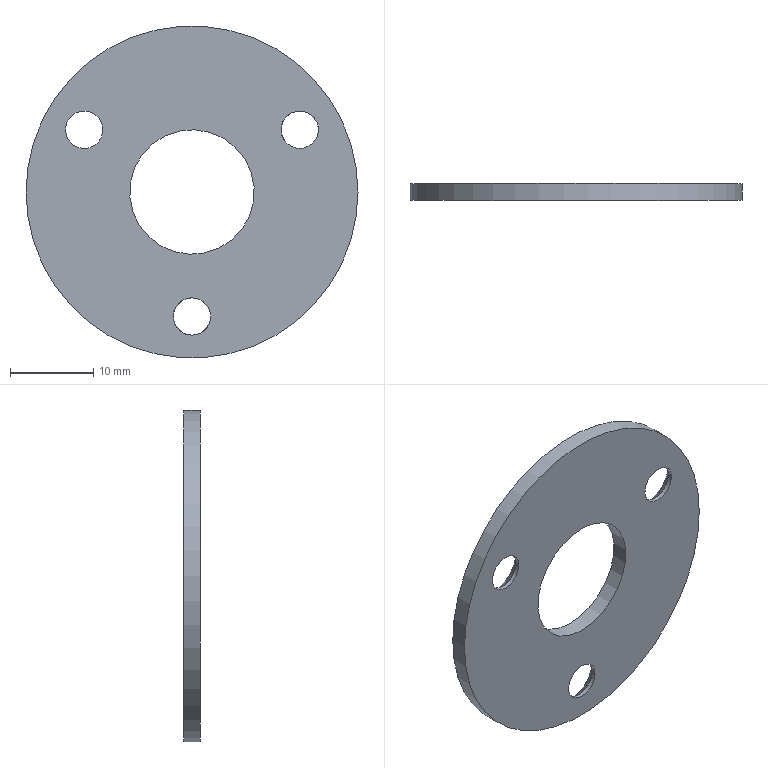Component | NX | GLAND | 1 solid | 10 faces | box 40 x 2 x 40 mm | volume 2006 mm3 | cylinder 5 | cone 3 | plane 2 | commonest cylinder face diameters 4.5 x3 15 x1 40 x1
STEP:
#1=CARTESIAN_POINT('',(0.,0.,0.));
#2=DIRECTION('',(0.,0.,1.));
#3=DIRECTION('',(1.,0.,0.));
#4=AXIS2_PLACEMENT_3D('',#1,#2,#3);
#5=CARTESIAN_POINT('',(3.75,36.,10.995));
#6=VERTEX_POINT('',#5);
#7=CARTESIAN_POINT('',(-0.,36.,4.5));
#8=DIRECTION('',(0.,-1.,0.));
#9=DIRECTION('',(0.5,0.,0.866));
#10=AXIS2_PLACEMENT_3D('',#7,#8,#9);
#11=CIRCLE('',#10,7.5);
#12=CARTESIAN_POINT('',(-0.,36.,4.5));
#13=DIRECTION('',(0.,-1.,0.));
#14=DIRECTION('',(-0.5,0.,-0.866));
#15=AXIS2_PLACEMENT_3D('',#12,#13,#14);
#16=CYLINDRICAL_SURFACE('',#15,7.5);
#17=CARTESIAN_POINT('',(3.142,0.));
#18=DIRECTION('',(1.,0.));
#19=VECTOR('',#18,1.);
#20=LINE('',#17,#19);
#21=(GEOMETRIC_REPRESENTATION_CONTEXT(2)PARAMETRIC_REPRESENTATION_CONTEXT()REPRESENTATION_CONTEXT('',''));
#22=DEFINITIONAL_REPRESENTATION('',(#20),#21);
#23=PCURVE('',#16,#22);
#24=CARTESIAN_POINT('',(-6.495,36.,8.25));
#25=DIRECTION('',(0.,-1.,0.));
#26=DIRECTION('',(-0.5,0.,-0.866));
#27=AXIS2_PLACEMENT_3D('',#24,#25,#26);
#28=PLANE('',#27);
#29=CARTESIAN_POINT('',(-0.,7.5));
#30=DIRECTION('',(-1.,0.));
#31=AXIS2_PLACEMENT_2D('',#29,#30);
#32=CIRCLE('',#31,7.5);
#33=(GEOMETRIC_REPRESENTATION_CONTEXT(2)PARAMETRIC_REPRESENTATION_CONTEXT()REPRESENTATION_CONTEXT('',''));
#34=DEFINITIONAL_REPRESENTATION('',(#32),#33);
#35=PCURVE('',#28,#34);
#36=SURFACE_CURVE('',#11,(#23,#35),.PCURVE_S1.);
#37=EDGE_CURVE('',#6,#6,#36,.T.);
#38=ORIENTED_EDGE('',*,*,#37,.T.);
#39=CARTESIAN_POINT('',(3.75,34.,10.995));
#40=VERTEX_POINT('',#39);
#41=CARTESIAN_POINT('',(3.75,36.,10.995));
#42=CARTESIAN_POINT('',(3.75,34.,10.995));
#43=B_SPLINE_CURVE_WITH_KNOTS('',1,(#41,#42),.UNSPECIFIED.,.F.,.F.,(2,2),(0.,2.),.PIECEWISE_BEZIER_KNOTS.);
#44=CARTESIAN_POINT('',(9.425,0.));
#45=DIRECTION('',(0.,1.));
#46=VECTOR('',#45,1.);
#47=LINE('',#44,#46);
#48=(GEOMETRIC_REPRESENTATION_CONTEXT(2)PARAMETRIC_REPRESENTATION_CONTEXT()REPRESENTATION_CONTEXT('',''));
#49=DEFINITIONAL_REPRESENTATION('',(#47),#48);
#50=PCURVE('',#16,#49);
#51=CARTESIAN_POINT('',(3.142,0.));
#52=DIRECTION('',(0.,1.));
#53=VECTOR('',#52,1.);
#54=LINE('',#51,#53);
#55=(GEOMETRIC_REPRESENTATION_CONTEXT(2)PARAMETRIC_REPRESENTATION_CONTEXT()REPRESENTATION_CONTEXT('',''));
#56=DEFINITIONAL_REPRESENTATION('',(#54),#55);
#57=PCURVE('',#16,#56);
#58=SEAM_CURVE('',#43,(#50,#57),.PCURVE_S1.);
#59=EDGE_CURVE('',#6,#40,#58,.T.);
#60=ORIENTED_EDGE('',*,*,#59,.T.);
#61=CARTESIAN_POINT('',(-0.,34.,4.5));
#62=DIRECTION('',(0.,-1.,0.));
#63=DIRECTION('',(0.5,0.,0.866));
#64=AXIS2_PLACEMENT_3D('',#61,#62,#63);
#65=CIRCLE('',#64,7.5);
#66=CARTESIAN_POINT('',(3.142,2.));
#67=DIRECTION('',(1.,0.));
#68=VECTOR('',#67,1.);
#69=LINE('',#66,#68);
#70=(GEOMETRIC_REPRESENTATION_CONTEXT(2)PARAMETRIC_REPRESENTATION_CONTEXT()REPRESENTATION_CONTEXT('',''));
#71=DEFINITIONAL_REPRESENTATION('',(#69),#70);
#72=PCURVE('',#16,#71);
#73=CARTESIAN_POINT('',(-6.495,34.,8.25));
#74=DIRECTION('',(0.,-1.,0.));
#75=DIRECTION('',(-0.5,0.,-0.866));
#76=AXIS2_PLACEMENT_3D('',#73,#74,#75);
#77=PLANE('',#76);
#78=CARTESIAN_POINT('',(-0.,7.5));
#79=DIRECTION('',(-1.,0.));
#80=AXIS2_PLACEMENT_2D('',#78,#79);
#81=CIRCLE('',#80,7.5);
#82=(GEOMETRIC_REPRESENTATION_CONTEXT(2)PARAMETRIC_REPRESENTATION_CONTEXT()REPRESENTATION_CONTEXT('',''));
#83=DEFINITIONAL_REPRESENTATION('',(#81),#82);
#84=PCURVE('',#77,#83);
#85=SURFACE_CURVE('',#65,(#72,#84),.PCURVE_S1.);
#86=EDGE_CURVE('',#40,#40,#85,.T.);
#87=ORIENTED_EDGE('',*,*,#86,.F.);
#88=ORIENTED_EDGE('',*,*,#59,.F.);
#89=EDGE_LOOP('',(#38,#60,#87,#88));
#90=FACE_BOUND('',#89,.F.);
#91=ADVANCED_FACE('',(#90),#16,.F.);
#92=CARTESIAN_POINT('',(-1.125,34.5,-12.449));
#93=VERTEX_POINT('',#92);
#94=CARTESIAN_POINT('',(0.,34.5,-10.5));
#95=DIRECTION('',(0.,1.,0.));
#96=DIRECTION('',(-0.5,0.,-0.866));
#97=AXIS2_PLACEMENT_3D('',#94,#95,#96);
#98=CIRCLE('',#97,2.25);
#99=CARTESIAN_POINT('',(0.,36.,-10.5));
#100=DIRECTION('',(0.,-1.,0.));
#101=DIRECTION('',(-0.5,0.,-0.866));
#102=AXIS2_PLACEMENT_3D('',#99,#100,#101);
#103=CYLINDRICAL_SURFACE('',#102,2.25);
#104=CARTESIAN_POINT('',(6.283,1.5));
#105=DIRECTION('',(-1.,0.));
#106=VECTOR('',#105,1.);
#107=LINE('',#104,#106);
#108=(GEOMETRIC_REPRESENTATION_CONTEXT(2)PARAMETRIC_REPRESENTATION_CONTEXT()REPRESENTATION_CONTEXT('',''));
#109=DEFINITIONAL_REPRESENTATION('',(#107),#108);
#110=PCURVE('',#103,#109);
#111=CARTESIAN_POINT('',(0.,36.,-10.5));
#112=DIRECTION('',(0.,1.,0.));
#113=DIRECTION('',(0.5,0.,0.866));
#114=AXIS2_PLACEMENT_3D('',#111,#112,#113);
#115=CONICAL_SURFACE('',#114,3.75,0.7854);
#116=CARTESIAN_POINT('',(3.142,-1.5));
#117=DIRECTION('',(1.,0.));
#118=VECTOR('',#117,1.);
#119=LINE('',#116,#118);
#120=(GEOMETRIC_REPRESENTATION_CONTEXT(2)PARAMETRIC_REPRESENTATION_CONTEXT()REPRESENTATION_CONTEXT('',''));
#121=DEFINITIONAL_REPRESENTATION('',(#119),#120);
#122=PCURVE('',#115,#121);
#123=SURFACE_CURVE('',#98,(#110,#122),.PCURVE_S1.);
#124=EDGE_CURVE('',#93,#93,#123,.T.);
#125=ORIENTED_EDGE('',*,*,#124,.F.);
#126=CARTESIAN_POINT('',(-1.125,34.,-12.449));
#127=VERTEX_POINT('',#126);
#128=CARTESIAN_POINT('',(-1.125,34.5,-12.449));
#129=CARTESIAN_POINT('',(-1.125,34.,-12.449));
#130=B_SPLINE_CURVE_WITH_KNOTS('',1,(#128,#129),.UNSPECIFIED.,.F.,.F.,(2,2),(1.5,2.),.PIECEWISE_BEZIER_KNOTS.);
#131=CARTESIAN_POINT('',(6.283,0.));
#132=DIRECTION('',(0.,1.));
#133=VECTOR('',#132,1.);
#134=LINE('',#131,#133);
#135=(GEOMETRIC_REPRESENTATION_CONTEXT(2)PARAMETRIC_REPRESENTATION_CONTEXT()REPRESENTATION_CONTEXT('',''));
#136=DEFINITIONAL_REPRESENTATION('',(#134),#135);
#137=PCURVE('',#103,#136);
#138=CARTESIAN_POINT('',(0.,0.));
#139=DIRECTION('',(0.,1.));
#140=VECTOR('',#139,1.);
#141=LINE('',#138,#140);
#142=(GEOMETRIC_REPRESENTATION_CONTEXT(2)PARAMETRIC_REPRESENTATION_CONTEXT()REPRESENTATION_CONTEXT('',''));
#143=DEFINITIONAL_REPRESENTATION('',(#141),#142);
#144=PCURVE('',#103,#143);
#145=SEAM_CURVE('',#130,(#137,#144),.PCURVE_S1.);
#146=EDGE_CURVE('',#93,#127,#145,.T.);
#147=ORIENTED_EDGE('',*,*,#146,.T.);
#148=CARTESIAN_POINT('',(-2.25,34.,-10.5));
#149=VERTEX_POINT('',#148);
#150=CARTESIAN_POINT('',(0.,34.,-10.5));
#151=DIRECTION('',(0.,-1.,0.));
#152=DIRECTION('',(-1.,0.,-0.));
#153=AXIS2_PLACEMENT_3D('',#150,#151,#152);
#154=CIRCLE('',#153,2.25);
#155=CARTESIAN_POINT('',(5.236,2.));
#156=DIRECTION('',(1.,0.));
#157=VECTOR('',#156,1.);
#158=LINE('',#155,#157);
#159=(GEOMETRIC_REPRESENTATION_CONTEXT(2)PARAMETRIC_REPRESENTATION_CONTEXT()REPRESENTATION_CONTEXT('',''));
#160=DEFINITIONAL_REPRESENTATION('',(#158),#159);
#161=PCURVE('',#103,#160);
#162=CARTESIAN_POINT('',(12.99,15.));
#163=DIRECTION('',(0.5,-0.866));
#164=AXIS2_PLACEMENT_2D('',#162,#163);
#165=CIRCLE('',#164,2.25);
#166=(GEOMETRIC_REPRESENTATION_CONTEXT(2)PARAMETRIC_REPRESENTATION_CONTEXT()REPRESENTATION_CONTEXT('',''));
#167=DEFINITIONAL_REPRESENTATION('',(#165),#166);
#168=PCURVE('',#77,#167);
#169=SURFACE_CURVE('',#154,(#161,#168),.PCURVE_S1.);
#170=EDGE_CURVE('',#149,#127,#169,.T.);
#171=ORIENTED_EDGE('',*,*,#170,.F.);
#172=CARTESIAN_POINT('',(0.,34.,-10.5));
#173=DIRECTION('',(0.,-1.,0.));
#174=DIRECTION('',(-1.,0.,-0.));
#175=AXIS2_PLACEMENT_3D('',#172,#173,#174);
#176=CIRCLE('',#175,2.25);
#177=CARTESIAN_POINT('',(-1.047,2.));
#178=DIRECTION('',(1.,0.));
#179=VECTOR('',#178,1.);
#180=LINE('',#177,#179);
#181=(GEOMETRIC_REPRESENTATION_CONTEXT(2)PARAMETRIC_REPRESENTATION_CONTEXT()REPRESENTATION_CONTEXT('',''));
#182=DEFINITIONAL_REPRESENTATION('',(#180),#181);
#183=PCURVE('',#103,#182);
#184=CARTESIAN_POINT('',(12.99,15.));
#185=DIRECTION('',(0.5,-0.866));
#186=AXIS2_PLACEMENT_2D('',#184,#185);
#187=CIRCLE('',#186,2.25);
#188=(GEOMETRIC_REPRESENTATION_CONTEXT(2)PARAMETRIC_REPRESENTATION_CONTEXT()REPRESENTATION_CONTEXT('',''));
#189=DEFINITIONAL_REPRESENTATION('',(#187),#188);
#190=PCURVE('',#77,#189);
#191=SURFACE_CURVE('',#176,(#183,#190),.PCURVE_S1.);
#192=EDGE_CURVE('',#127,#149,#191,.T.);
#193=ORIENTED_EDGE('',*,*,#192,.F.);
#194=ORIENTED_EDGE('',*,*,#146,.F.);
#195=EDGE_LOOP('',(#125,#147,#171,#193,#194));
#196=FACE_BOUND('',#195,.F.);
#197=ADVANCED_FACE('',(#196),#103,.F.);
#198=CARTESIAN_POINT('',(-14.115,34.5,10.051));
#199=VERTEX_POINT('',#198);
#200=CARTESIAN_POINT('',(-12.99,34.5,12.));
#201=DIRECTION('',(0.,1.,0.));
#202=DIRECTION('',(-0.5,0.,-0.866));
#203=AXIS2_PLACEMENT_3D('',#200,#201,#202);
#204=CIRCLE('',#203,2.25);
#205=CARTESIAN_POINT('',(-12.99,36.,12.));
#206=DIRECTION('',(0.,-1.,0.));
#207=DIRECTION('',(-0.5,0.,-0.866));
#208=AXIS2_PLACEMENT_3D('',#205,#206,#207);
#209=CYLINDRICAL_SURFACE('',#208,2.25);
#210=CARTESIAN_POINT('',(6.283,1.5));
#211=DIRECTION('',(-1.,0.));
#212=VECTOR('',#211,1.);
#213=LINE('',#210,#212);
#214=(GEOMETRIC_REPRESENTATION_CONTEXT(2)PARAMETRIC_REPRESENTATION_CONTEXT()REPRESENTATION_CONTEXT('',''));
#215=DEFINITIONAL_REPRESENTATION('',(#213),#214);
#216=PCURVE('',#209,#215);
#217=CARTESIAN_POINT('',(-12.99,36.,12.));
#218=DIRECTION('',(0.,1.,0.));
#219=DIRECTION('',(0.5,0.,0.866));
#220=AXIS2_PLACEMENT_3D('',#217,#218,#219);
#221=CONICAL_SURFACE('',#220,3.75,0.7854);
#222=CARTESIAN_POINT('',(3.142,-1.5));
#223=DIRECTION('',(1.,0.));
#224=VECTOR('',#223,1.);
#225=LINE('',#222,#224);
#226=(GEOMETRIC_REPRESENTATION_CONTEXT(2)PARAMETRIC_REPRESENTATION_CONTEXT()REPRESENTATION_CONTEXT('',''));
#227=DEFINITIONAL_REPRESENTATION('',(#225),#226);
#228=PCURVE('',#221,#227);
#229=SURFACE_CURVE('',#204,(#216,#228),.PCURVE_S1.);
#230=EDGE_CURVE('',#199,#199,#229,.T.);
#231=ORIENTED_EDGE('',*,*,#230,.F.);
#232=CARTESIAN_POINT('',(-14.115,34.,10.051));
#233=VERTEX_POINT('',#232);
#234=CARTESIAN_POINT('',(-14.115,34.5,10.051));
#235=CARTESIAN_POINT('',(-14.115,34.,10.051));
#236=B_SPLINE_CURVE_WITH_KNOTS('',1,(#234,#235),.UNSPECIFIED.,.F.,.F.,(2,2),(1.5,2.),.PIECEWISE_BEZIER_KNOTS.);
#237=CARTESIAN_POINT('',(6.283,0.));
#238=DIRECTION('',(0.,1.));
#239=VECTOR('',#238,1.);
#240=LINE('',#237,#239);
#241=(GEOMETRIC_REPRESENTATION_CONTEXT(2)PARAMETRIC_REPRESENTATION_CONTEXT()REPRESENTATION_CONTEXT('',''));
#242=DEFINITIONAL_REPRESENTATION('',(#240),#241);
#243=PCURVE('',#209,#242);
#244=CARTESIAN_POINT('',(0.,0.));
#245=DIRECTION('',(0.,1.));
#246=VECTOR('',#245,1.);
#247=LINE('',#244,#246);
#248=(GEOMETRIC_REPRESENTATION_CONTEXT(2)PARAMETRIC_REPRESENTATION_CONTEXT()REPRESENTATION_CONTEXT('',''));
#249=DEFINITIONAL_REPRESENTATION('',(#247),#248);
#250=PCURVE('',#209,#249);
#251=SEAM_CURVE('',#236,(#243,#250),.PCURVE_S1.);
#252=EDGE_CURVE('',#199,#233,#251,.T.);
#253=ORIENTED_EDGE('',*,*,#252,.T.);
#254=CARTESIAN_POINT('',(-11.865,34.,13.949));
#255=VERTEX_POINT('',#254);
#256=CARTESIAN_POINT('',(-12.99,34.,12.));
#257=DIRECTION('',(0.,-1.,0.));
#258=DIRECTION('',(0.5,0.,0.866));
#259=AXIS2_PLACEMENT_3D('',#256,#257,#258);
#260=CIRCLE('',#259,2.25);
#261=CARTESIAN_POINT('',(3.142,2.));
#262=DIRECTION('',(1.,0.));
#263=VECTOR('',#262,1.);
#264=LINE('',#261,#263);
#265=(GEOMETRIC_REPRESENTATION_CONTEXT(2)PARAMETRIC_REPRESENTATION_CONTEXT()REPRESENTATION_CONTEXT('',''));
#266=DEFINITIONAL_REPRESENTATION('',(#264),#265);
#267=PCURVE('',#209,#266);
#268=CARTESIAN_POINT('',(-0.,-7.5));
#269=DIRECTION('',(-1.,0.));
#270=AXIS2_PLACEMENT_2D('',#268,#269);
#271=CIRCLE('',#270,2.25);
#272=(GEOMETRIC_REPRESENTATION_CONTEXT(2)PARAMETRIC_REPRESENTATION_CONTEXT()REPRESENTATION_CONTEXT('',''));
#273=DEFINITIONAL_REPRESENTATION('',(#271),#272);
#274=PCURVE('',#77,#273);
#275=SURFACE_CURVE('',#260,(#267,#274),.PCURVE_S1.);
#276=EDGE_CURVE('',#255,#233,#275,.T.);
#277=ORIENTED_EDGE('',*,*,#276,.F.);
#278=CARTESIAN_POINT('',(-12.99,34.,12.));
#279=DIRECTION('',(0.,-1.,0.));
#280=DIRECTION('',(0.5,0.,0.866));
#281=AXIS2_PLACEMENT_3D('',#278,#279,#280);
#282=CIRCLE('',#281,2.25);
#283=CARTESIAN_POINT('',(-3.142,2.));
#284=DIRECTION('',(1.,0.));
#285=VECTOR('',#284,1.);
#286=LINE('',#283,#285);
#287=(GEOMETRIC_REPRESENTATION_CONTEXT(2)PARAMETRIC_REPRESENTATION_CONTEXT()REPRESENTATION_CONTEXT('',''));
#288=DEFINITIONAL_REPRESENTATION('',(#286),#287);
#289=PCURVE('',#209,#288);
#290=CARTESIAN_POINT('',(-0.,-7.5));
#291=DIRECTION('',(-1.,0.));
#292=AXIS2_PLACEMENT_2D('',#290,#291);
#293=CIRCLE('',#292,2.25);
#294=(GEOMETRIC_REPRESENTATION_CONTEXT(2)PARAMETRIC_REPRESENTATION_CONTEXT()REPRESENTATION_CONTEXT('',''));
#295=DEFINITIONAL_REPRESENTATION('',(#293),#294);
#296=PCURVE('',#77,#295);
#297=SURFACE_CURVE('',#282,(#289,#296),.PCURVE_S1.);
#298=EDGE_CURVE('',#233,#255,#297,.T.);
#299=ORIENTED_EDGE('',*,*,#298,.F.);
#300=ORIENTED_EDGE('',*,*,#252,.F.);
#301=EDGE_LOOP('',(#231,#253,#277,#299,#300));
#302=FACE_BOUND('',#301,.F.);
#303=ADVANCED_FACE('',(#302),#209,.F.);
#304=CARTESIAN_POINT('',(10.,36.,21.821));
#305=VERTEX_POINT('',#304);
#306=CARTESIAN_POINT('',(-0.,36.,4.5));
#307=DIRECTION('',(0.,-1.,0.));
#308=DIRECTION('',(0.5,0.,0.866));
#309=AXIS2_PLACEMENT_3D('',#306,#307,#308);
#310=CIRCLE('',#309,20.);
#311=CARTESIAN_POINT('',(-0.,36.,4.5));
#312=DIRECTION('',(0.,-1.,0.));
#313=DIRECTION('',(-0.5,0.,-0.866));
#314=AXIS2_PLACEMENT_3D('',#311,#312,#313);
#315=CYLINDRICAL_SURFACE('',#314,20.);
#316=CARTESIAN_POINT('',(3.142,0.));
#317=DIRECTION('',(1.,0.));
#318=VECTOR('',#317,1.);
#319=LINE('',#316,#318);
#320=(GEOMETRIC_REPRESENTATION_CONTEXT(2)PARAMETRIC_REPRESENTATION_CONTEXT()REPRESENTATION_CONTEXT('',''));
#321=DEFINITIONAL_REPRESENTATION('',(#319),#320);
#322=PCURVE('',#315,#321);
#323=CARTESIAN_POINT('',(-0.,7.5));
#324=DIRECTION('',(-1.,0.));
#325=AXIS2_PLACEMENT_2D('',#323,#324);
#326=CIRCLE('',#325,20.);
#327=(GEOMETRIC_REPRESENTATION_CONTEXT(2)PARAMETRIC_REPRESENTATION_CONTEXT()REPRESENTATION_CONTEXT('',''));
#328=DEFINITIONAL_REPRESENTATION('',(#326),#327);
#329=PCURVE('',#28,#328);
#330=SURFACE_CURVE('',#310,(#322,#329),.PCURVE_S1.);
#331=EDGE_CURVE('',#305,#305,#330,.T.);
#332=ORIENTED_EDGE('',*,*,#331,.T.);
#333=CARTESIAN_POINT('',(10.,34.,21.821));
#334=VERTEX_POINT('',#333);
#335=CARTESIAN_POINT('',(10.,36.,21.821));
#336=CARTESIAN_POINT('',(10.,34.,21.821));
#337=B_SPLINE_CURVE_WITH_KNOTS('',1,(#335,#336),.UNSPECIFIED.,.F.,.F.,(2,2),(0.,2.),.PIECEWISE_BEZIER_KNOTS.);
#338=CARTESIAN_POINT('',(9.425,0.));
#339=DIRECTION('',(0.,1.));
#340=VECTOR('',#339,1.);
#341=LINE('',#338,#340);
#342=(GEOMETRIC_REPRESENTATION_CONTEXT(2)PARAMETRIC_REPRESENTATION_CONTEXT()REPRESENTATION_CONTEXT('',''));
#343=DEFINITIONAL_REPRESENTATION('',(#341),#342);
#344=PCURVE('',#315,#343);
#345=CARTESIAN_POINT('',(3.142,0.));
#346=DIRECTION('',(0.,1.));
#347=VECTOR('',#346,1.);
#348=LINE('',#345,#347);
#349=(GEOMETRIC_REPRESENTATION_CONTEXT(2)PARAMETRIC_REPRESENTATION_CONTEXT()REPRESENTATION_CONTEXT('',''));
#350=DEFINITIONAL_REPRESENTATION('',(#348),#349);
#351=PCURVE('',#315,#350);
#352=SEAM_CURVE('',#337,(#344,#351),.PCURVE_S1.);
#353=EDGE_CURVE('',#305,#334,#352,.T.);
#354=ORIENTED_EDGE('',*,*,#353,.T.);
#355=CARTESIAN_POINT('',(-0.,34.,4.5));
#356=DIRECTION('',(0.,-1.,0.));
#357=DIRECTION('',(0.5,0.,0.866));
#358=AXIS2_PLACEMENT_3D('',#355,#356,#357);
#359=CIRCLE('',#358,20.);
#360=CARTESIAN_POINT('',(3.142,2.));
#361=DIRECTION('',(1.,0.));
#362=VECTOR('',#361,1.);
#363=LINE('',#360,#362);
#364=(GEOMETRIC_REPRESENTATION_CONTEXT(2)PARAMETRIC_REPRESENTATION_CONTEXT()REPRESENTATION_CONTEXT('',''));
#365=DEFINITIONAL_REPRESENTATION('',(#363),#364);
#366=PCURVE('',#315,#365);
#367=CARTESIAN_POINT('',(-0.,7.5));
#368=DIRECTION('',(-1.,0.));
#369=AXIS2_PLACEMENT_2D('',#367,#368);
#370=CIRCLE('',#369,20.);
#371=(GEOMETRIC_REPRESENTATION_CONTEXT(2)PARAMETRIC_REPRESENTATION_CONTEXT()REPRESENTATION_CONTEXT('',''));
#372=DEFINITIONAL_REPRESENTATION('',(#370),#371);
#373=PCURVE('',#77,#372);
#374=SURFACE_CURVE('',#359,(#366,#373),.PCURVE_S1.);
#375=EDGE_CURVE('',#334,#334,#374,.T.);
#376=ORIENTED_EDGE('',*,*,#375,.F.);
#377=ORIENTED_EDGE('',*,*,#353,.F.);
#378=EDGE_LOOP('',(#332,#354,#376,#377));
#379=FACE_BOUND('',#378,.T.);
#380=ADVANCED_FACE('',(#379),#315,.T.);
#381=CARTESIAN_POINT('',(11.865,34.5,10.051));
#382=VERTEX_POINT('',#381);
#383=CARTESIAN_POINT('',(12.99,34.5,12.));
#384=DIRECTION('',(0.,1.,0.));
#385=DIRECTION('',(-0.5,0.,-0.866));
#386=AXIS2_PLACEMENT_3D('',#383,#384,#385);
#387=CIRCLE('',#386,2.25);
#388=CARTESIAN_POINT('',(12.99,36.,12.));
#389=DIRECTION('',(0.,-1.,0.));
#390=DIRECTION('',(-0.5,0.,-0.866));
#391=AXIS2_PLACEMENT_3D('',#388,#389,#390);
#392=CYLINDRICAL_SURFACE('',#391,2.25);
#393=CARTESIAN_POINT('',(6.283,1.5));
#394=DIRECTION('',(-1.,0.));
#395=VECTOR('',#394,1.);
#396=LINE('',#393,#395);
#397=(GEOMETRIC_REPRESENTATION_CONTEXT(2)PARAMETRIC_REPRESENTATION_CONTEXT()REPRESENTATION_CONTEXT('',''));
#398=DEFINITIONAL_REPRESENTATION('',(#396),#397);
#399=PCURVE('',#392,#398);
#400=CARTESIAN_POINT('',(12.99,36.,12.));
#401=DIRECTION('',(0.,1.,0.));
#402=DIRECTION('',(0.5,0.,0.866));
#403=AXIS2_PLACEMENT_3D('',#400,#401,#402);
#404=CONICAL_SURFACE('',#403,3.75,0.7854);
#405=CARTESIAN_POINT('',(3.142,-1.5));
#406=DIRECTION('',(1.,0.));
#407=VECTOR('',#406,1.);
#408=LINE('',#405,#407);
#409=(GEOMETRIC_REPRESENTATION_CONTEXT(2)PARAMETRIC_REPRESENTATION_CONTEXT()REPRESENTATION_CONTEXT('',''));
#410=DEFINITIONAL_REPRESENTATION('',(#408),#409);
#411=PCURVE('',#404,#410);
#412=SURFACE_CURVE('',#387,(#399,#411),.PCURVE_S1.);
#413=EDGE_CURVE('',#382,#382,#412,.T.);
#414=ORIENTED_EDGE('',*,*,#413,.F.);
#415=CARTESIAN_POINT('',(11.865,34.,10.051));
#416=VERTEX_POINT('',#415);
#417=CARTESIAN_POINT('',(11.865,34.5,10.051));
#418=CARTESIAN_POINT('',(11.865,34.,10.051));
#419=B_SPLINE_CURVE_WITH_KNOTS('',1,(#417,#418),.UNSPECIFIED.,.F.,.F.,(2,2),(1.5,2.),.PIECEWISE_BEZIER_KNOTS.);
#420=CARTESIAN_POINT('',(6.283,0.));
#421=DIRECTION('',(0.,1.));
#422=VECTOR('',#421,1.);
#423=LINE('',#420,#422);
#424=(GEOMETRIC_REPRESENTATION_CONTEXT(2)PARAMETRIC_REPRESENTATION_CONTEXT()REPRESENTATION_CONTEXT('',''));
#425=DEFINITIONAL_REPRESENTATION('',(#423),#424);
#426=PCURVE('',#392,#425);
#427=CARTESIAN_POINT('',(0.,0.));
#428=DIRECTION('',(0.,1.));
#429=VECTOR('',#428,1.);
#430=LINE('',#427,#429);
#431=(GEOMETRIC_REPRESENTATION_CONTEXT(2)PARAMETRIC_REPRESENTATION_CONTEXT()REPRESENTATION_CONTEXT('',''));
#432=DEFINITIONAL_REPRESENTATION('',(#430),#431);
#433=PCURVE('',#392,#432);
#434=SEAM_CURVE('',#419,(#426,#433),.PCURVE_S1.);
#435=EDGE_CURVE('',#382,#416,#434,.T.);
#436=ORIENTED_EDGE('',*,*,#435,.T.);
#437=CARTESIAN_POINT('',(14.115,34.,10.051));
#438=VERTEX_POINT('',#437);
#439=CARTESIAN_POINT('',(12.99,34.,12.));
#440=DIRECTION('',(0.,-1.,0.));
#441=DIRECTION('',(0.5,0.,-0.866));
#442=AXIS2_PLACEMENT_3D('',#439,#440,#441);
#443=CIRCLE('',#442,2.25);
#444=CARTESIAN_POINT('',(1.047,2.));
#445=DIRECTION('',(1.,0.));
#446=VECTOR('',#445,1.);
#447=LINE('',#444,#446);
#448=(GEOMETRIC_REPRESENTATION_CONTEXT(2)PARAMETRIC_REPRESENTATION_CONTEXT()REPRESENTATION_CONTEXT('',''));
#449=DEFINITIONAL_REPRESENTATION('',(#447),#448);
#450=PCURVE('',#392,#449);
#451=CARTESIAN_POINT('',(-12.99,15.));
#452=DIRECTION('',(0.5,0.866));
#453=AXIS2_PLACEMENT_2D('',#451,#452);
#454=CIRCLE('',#453,2.25);
#455=(GEOMETRIC_REPRESENTATION_CONTEXT(2)PARAMETRIC_REPRESENTATION_CONTEXT()REPRESENTATION_CONTEXT('',''));
#456=DEFINITIONAL_REPRESENTATION('',(#454),#455);
#457=PCURVE('',#77,#456);
#458=SURFACE_CURVE('',#443,(#450,#457),.PCURVE_S1.);
#459=EDGE_CURVE('',#438,#416,#458,.T.);
#460=ORIENTED_EDGE('',*,*,#459,.F.);
#461=CARTESIAN_POINT('',(12.99,34.,12.));
#462=DIRECTION('',(0.,-1.,0.));
#463=DIRECTION('',(0.5,0.,-0.866));
#464=AXIS2_PLACEMENT_3D('',#461,#462,#463);
#465=CIRCLE('',#464,2.25);
#466=CARTESIAN_POINT('',(-5.236,2.));
#467=DIRECTION('',(1.,0.));
#468=VECTOR('',#467,1.);
#469=LINE('',#466,#468);
#470=(GEOMETRIC_REPRESENTATION_CONTEXT(2)PARAMETRIC_REPRESENTATION_CONTEXT()REPRESENTATION_CONTEXT('',''));
#471=DEFINITIONAL_REPRESENTATION('',(#469),#470);
#472=PCURVE('',#392,#471);
#473=CARTESIAN_POINT('',(-12.99,15.));
#474=DIRECTION('',(0.5,0.866));
#475=AXIS2_PLACEMENT_2D('',#473,#474);
#476=CIRCLE('',#475,2.25);
#477=(GEOMETRIC_REPRESENTATION_CONTEXT(2)PARAMETRIC_REPRESENTATION_CONTEXT()REPRESENTATION_CONTEXT('',''));
#478=DEFINITIONAL_REPRESENTATION('',(#476),#477);
#479=PCURVE('',#77,#478);
#480=SURFACE_CURVE('',#465,(#472,#479),.PCURVE_S1.);
#481=EDGE_CURVE('',#416,#438,#480,.T.);
#482=ORIENTED_EDGE('',*,*,#481,.F.);
#483=ORIENTED_EDGE('',*,*,#435,.F.);
#484=EDGE_LOOP('',(#414,#436,#460,#482,#483));
#485=FACE_BOUND('',#484,.F.);
#486=ADVANCED_FACE('',(#485),#392,.F.);
#487=CARTESIAN_POINT('',(-1.875,36.,-13.748));
#488=VERTEX_POINT('',#487);
#489=CARTESIAN_POINT('',(0.,36.,-10.5));
#490=DIRECTION('',(0.,-1.,0.));
#491=DIRECTION('',(-0.5,0.,-0.866));
#492=AXIS2_PLACEMENT_3D('',#489,#490,#491);
#493=CIRCLE('',#492,3.75);
#494=CARTESIAN_POINT('',(12.99,15.));
#495=DIRECTION('',(1.,0.));
#496=AXIS2_PLACEMENT_2D('',#494,#495);
#497=CIRCLE('',#496,3.75);
#498=(GEOMETRIC_REPRESENTATION_CONTEXT(2)PARAMETRIC_REPRESENTATION_CONTEXT()REPRESENTATION_CONTEXT('',''));
#499=DEFINITIONAL_REPRESENTATION('',(#497),#498);
#500=PCURVE('',#28,#499);
#501=CARTESIAN_POINT('',(9.425,0.));
#502=DIRECTION('',(-1.,0.));
#503=VECTOR('',#502,1.);
#504=LINE('',#501,#503);
#505=(GEOMETRIC_REPRESENTATION_CONTEXT(2)PARAMETRIC_REPRESENTATION_CONTEXT()REPRESENTATION_CONTEXT('',''));
#506=DEFINITIONAL_REPRESENTATION('',(#504),#505);
#507=PCURVE('',#115,#506);
#508=SURFACE_CURVE('',#493,(#500,#507),.PCURVE_S1.);
#509=EDGE_CURVE('',#488,#488,#508,.T.);
#510=ORIENTED_EDGE('',*,*,#509,.T.);
#511=EDGE_LOOP('',(#510));
#512=FACE_BOUND('',#511,.T.);
#513=CARTESIAN_POINT('',(11.115,36.,8.752));
#514=VERTEX_POINT('',#513);
#515=CARTESIAN_POINT('',(12.99,36.,12.));
#516=DIRECTION('',(0.,-1.,0.));
#517=DIRECTION('',(-0.5,0.,-0.866));
#518=AXIS2_PLACEMENT_3D('',#515,#516,#517);
#519=CIRCLE('',#518,3.75);
#520=CARTESIAN_POINT('',(-12.99,15.));
#521=DIRECTION('',(1.,0.));
#522=AXIS2_PLACEMENT_2D('',#520,#521);
#523=CIRCLE('',#522,3.75);
#524=(GEOMETRIC_REPRESENTATION_CONTEXT(2)PARAMETRIC_REPRESENTATION_CONTEXT()REPRESENTATION_CONTEXT('',''));
#525=DEFINITIONAL_REPRESENTATION('',(#523),#524);
#526=PCURVE('',#28,#525);
#527=CARTESIAN_POINT('',(9.425,0.));
#528=DIRECTION('',(-1.,0.));
#529=VECTOR('',#528,1.);
#530=LINE('',#527,#529);
#531=(GEOMETRIC_REPRESENTATION_CONTEXT(2)PARAMETRIC_REPRESENTATION_CONTEXT()REPRESENTATION_CONTEXT('',''));
#532=DEFINITIONAL_REPRESENTATION('',(#530),#531);
#533=PCURVE('',#404,#532);
#534=SURFACE_CURVE('',#519,(#526,#533),.PCURVE_S1.);
#535=EDGE_CURVE('',#514,#514,#534,.T.);
#536=ORIENTED_EDGE('',*,*,#535,.T.);
#537=EDGE_LOOP('',(#536));
#538=FACE_BOUND('',#537,.T.);
#539=CARTESIAN_POINT('',(-14.865,36.,8.752));
#540=VERTEX_POINT('',#539);
#541=CARTESIAN_POINT('',(-12.99,36.,12.));
#542=DIRECTION('',(0.,-1.,0.));
#543=DIRECTION('',(-0.5,0.,-0.866));
#544=AXIS2_PLACEMENT_3D('',#541,#542,#543);
#545=CIRCLE('',#544,3.75);
#546=CARTESIAN_POINT('',(-0.,-7.5));
#547=DIRECTION('',(1.,0.));
#548=AXIS2_PLACEMENT_2D('',#546,#547);
#549=CIRCLE('',#548,3.75);
#550=(GEOMETRIC_REPRESENTATION_CONTEXT(2)PARAMETRIC_REPRESENTATION_CONTEXT()REPRESENTATION_CONTEXT('',''));
#551=DEFINITIONAL_REPRESENTATION('',(#549),#550);
#552=PCURVE('',#28,#551);
#553=CARTESIAN_POINT('',(9.425,0.));
#554=DIRECTION('',(-1.,0.));
#555=VECTOR('',#554,1.);
#556=LINE('',#553,#555);
#557=(GEOMETRIC_REPRESENTATION_CONTEXT(2)PARAMETRIC_REPRESENTATION_CONTEXT()REPRESENTATION_CONTEXT('',''));
#558=DEFINITIONAL_REPRESENTATION('',(#556),#557);
#559=PCURVE('',#221,#558);
#560=SURFACE_CURVE('',#545,(#552,#559),.PCURVE_S1.);
#561=EDGE_CURVE('',#540,#540,#560,.T.);
#562=ORIENTED_EDGE('',*,*,#561,.T.);
#563=EDGE_LOOP('',(#562));
#564=FACE_BOUND('',#563,.T.);
#565=ORIENTED_EDGE('',*,*,#331,.F.);
#566=EDGE_LOOP('',(#565));
#567=FACE_BOUND('',#566,.T.);
#568=ORIENTED_EDGE('',*,*,#37,.T.);
#569=EDGE_LOOP('',(#568));
#570=FACE_BOUND('',#569,.T.);
#571=ADVANCED_FACE('',(#512,#538,#564,#567,#570),#28,.F.);
#572=ORIENTED_EDGE('',*,*,#375,.T.);
#573=EDGE_LOOP('',(#572));
#574=FACE_BOUND('',#573,.T.);
#575=ORIENTED_EDGE('',*,*,#276,.F.);
#576=ORIENTED_EDGE('',*,*,#298,.F.);
#577=EDGE_LOOP('',(#575,#576));
#578=FACE_BOUND('',#577,.T.);
#579=ORIENTED_EDGE('',*,*,#170,.F.);
#580=ORIENTED_EDGE('',*,*,#192,.F.);
#581=EDGE_LOOP('',(#579,#580));
#582=FACE_BOUND('',#581,.T.);
#583=ORIENTED_EDGE('',*,*,#86,.F.);
#584=EDGE_LOOP('',(#583));
#585=FACE_BOUND('',#584,.T.);
#586=ORIENTED_EDGE('',*,*,#459,.F.);
#587=ORIENTED_EDGE('',*,*,#481,.F.);
#588=EDGE_LOOP('',(#586,#587));
#589=FACE_BOUND('',#588,.T.);
#590=ADVANCED_FACE('',(#574,#578,#582,#585,#589),#77,.T.);
#591=ORIENTED_EDGE('',*,*,#124,.T.);
#592=CARTESIAN_POINT('',(-1.125,34.5,-12.449));
#593=CARTESIAN_POINT('',(-1.875,36.,-13.748));
#594=B_SPLINE_CURVE_WITH_KNOTS('',1,(#592,#593),.UNSPECIFIED.,.F.,.F.,(2,2),(-2.121,0.),.PIECEWISE_BEZIER_KNOTS.);
#595=CARTESIAN_POINT('',(9.425,0.));
#596=DIRECTION('',(0.,1.));
#597=VECTOR('',#596,1.);
#598=LINE('',#595,#597);
#599=(GEOMETRIC_REPRESENTATION_CONTEXT(2)PARAMETRIC_REPRESENTATION_CONTEXT()REPRESENTATION_CONTEXT('',''));
#600=DEFINITIONAL_REPRESENTATION('',(#598),#599);
#601=PCURVE('',#115,#600);
#602=CARTESIAN_POINT('',(3.142,0.));
#603=DIRECTION('',(0.,1.));
#604=VECTOR('',#603,1.);
#605=LINE('',#602,#604);
#606=(GEOMETRIC_REPRESENTATION_CONTEXT(2)PARAMETRIC_REPRESENTATION_CONTEXT()REPRESENTATION_CONTEXT('',''));
#607=DEFINITIONAL_REPRESENTATION('',(#605),#606);
#608=PCURVE('',#115,#607);
#609=SEAM_CURVE('',#594,(#601,#608),.PCURVE_S1.);
#610=EDGE_CURVE('',#93,#488,#609,.T.);
#611=ORIENTED_EDGE('',*,*,#610,.T.);
#612=ORIENTED_EDGE('',*,*,#509,.T.);
#613=ORIENTED_EDGE('',*,*,#610,.F.);
#614=EDGE_LOOP('',(#591,#611,#612,#613));
#615=FACE_BOUND('',#614,.F.);
#616=ADVANCED_FACE('',(#615),#115,.F.);
#617=ORIENTED_EDGE('',*,*,#413,.T.);
#618=CARTESIAN_POINT('',(11.865,34.5,10.051));
#619=CARTESIAN_POINT('',(11.115,36.,8.752));
#620=B_SPLINE_CURVE_WITH_KNOTS('',1,(#618,#619),.UNSPECIFIED.,.F.,.F.,(2,2),(-2.121,0.),.PIECEWISE_BEZIER_KNOTS.);
#621=CARTESIAN_POINT('',(9.425,0.));
#622=DIRECTION('',(0.,1.));
#623=VECTOR('',#622,1.);
#624=LINE('',#621,#623);
#625=(GEOMETRIC_REPRESENTATION_CONTEXT(2)PARAMETRIC_REPRESENTATION_CONTEXT()REPRESENTATION_CONTEXT('',''));
#626=DEFINITIONAL_REPRESENTATION('',(#624),#625);
#627=PCURVE('',#404,#626);
#628=CARTESIAN_POINT('',(3.142,0.));
#629=DIRECTION('',(0.,1.));
#630=VECTOR('',#629,1.);
#631=LINE('',#628,#630);
#632=(GEOMETRIC_REPRESENTATION_CONTEXT(2)PARAMETRIC_REPRESENTATION_CONTEXT()REPRESENTATION_CONTEXT('',''));
#633=DEFINITIONAL_REPRESENTATION('',(#631),#632);
#634=PCURVE('',#404,#633);
#635=SEAM_CURVE('',#620,(#627,#634),.PCURVE_S1.);
#636=EDGE_CURVE('',#382,#514,#635,.T.);
#637=ORIENTED_EDGE('',*,*,#636,.T.);
#638=ORIENTED_EDGE('',*,*,#535,.T.);
#639=ORIENTED_EDGE('',*,*,#636,.F.);
#640=EDGE_LOOP('',(#617,#637,#638,#639));
#641=FACE_BOUND('',#640,.F.);
#642=ADVANCED_FACE('',(#641),#404,.F.);
#643=ORIENTED_EDGE('',*,*,#230,.T.);
#644=CARTESIAN_POINT('',(-14.115,34.5,10.051));
#645=CARTESIAN_POINT('',(-14.865,36.,8.752));
#646=B_SPLINE_CURVE_WITH_KNOTS('',1,(#644,#645),.UNSPECIFIED.,.F.,.F.,(2,2),(-2.121,0.),.PIECEWISE_BEZIER_KNOTS.);
#647=CARTESIAN_POINT('',(9.425,0.));
#648=DIRECTION('',(0.,1.));
#649=VECTOR('',#648,1.);
#650=LINE('',#647,#649);
#651=(GEOMETRIC_REPRESENTATION_CONTEXT(2)PARAMETRIC_REPRESENTATION_CONTEXT()REPRESENTATION_CONTEXT('',''));
#652=DEFINITIONAL_REPRESENTATION('',(#650),#651);
#653=PCURVE('',#221,#652);
#654=CARTESIAN_POINT('',(3.142,0.));
#655=DIRECTION('',(0.,1.));
#656=VECTOR('',#655,1.);
#657=LINE('',#654,#656);
#658=(GEOMETRIC_REPRESENTATION_CONTEXT(2)PARAMETRIC_REPRESENTATION_CONTEXT()REPRESENTATION_CONTEXT('',''));
#659=DEFINITIONAL_REPRESENTATION('',(#657),#658);
#660=PCURVE('',#221,#659);
#661=SEAM_CURVE('',#646,(#653,#660),.PCURVE_S1.);
#662=EDGE_CURVE('',#199,#540,#661,.T.);
#663=ORIENTED_EDGE('',*,*,#662,.T.);
#664=ORIENTED_EDGE('',*,*,#561,.T.);
#665=ORIENTED_EDGE('',*,*,#662,.F.);
#666=EDGE_LOOP('',(#643,#663,#664,#665));
#667=FACE_BOUND('',#666,.F.);
#668=ADVANCED_FACE('',(#667),#221,.F.);
#669=CLOSED_SHELL('',(#91,#197,#303,#380,#486,#571,#590,#616,#642,#668));
#670=MANIFOLD_SOLID_BREP('',#669);
#671=(LENGTH_UNIT()NAMED_UNIT(*)SI_UNIT(.MILLI.,.METRE.));
#672=UNCERTAINTY_MEASURE_WITH_UNIT(LENGTH_MEASURE(0.000005),#671,'','');
#673=(NAMED_UNIT(*)PLANE_ANGLE_UNIT()SI_UNIT($,.RADIAN.));
#674=(NAMED_UNIT(*)SI_UNIT($,.STERADIAN.)SOLID_ANGLE_UNIT());
#675=(GEOMETRIC_REPRESENTATION_CONTEXT(3)GLOBAL_UNCERTAINTY_ASSIGNED_CONTEXT((#672))GLOBAL_UNIT_ASSIGNED_CONTEXT((#671,#673,#674))REPRESENTATION_CONTEXT('',''));
#676=ADVANCED_BREP_SHAPE_REPRESENTATION('',(#4,#670),#675);